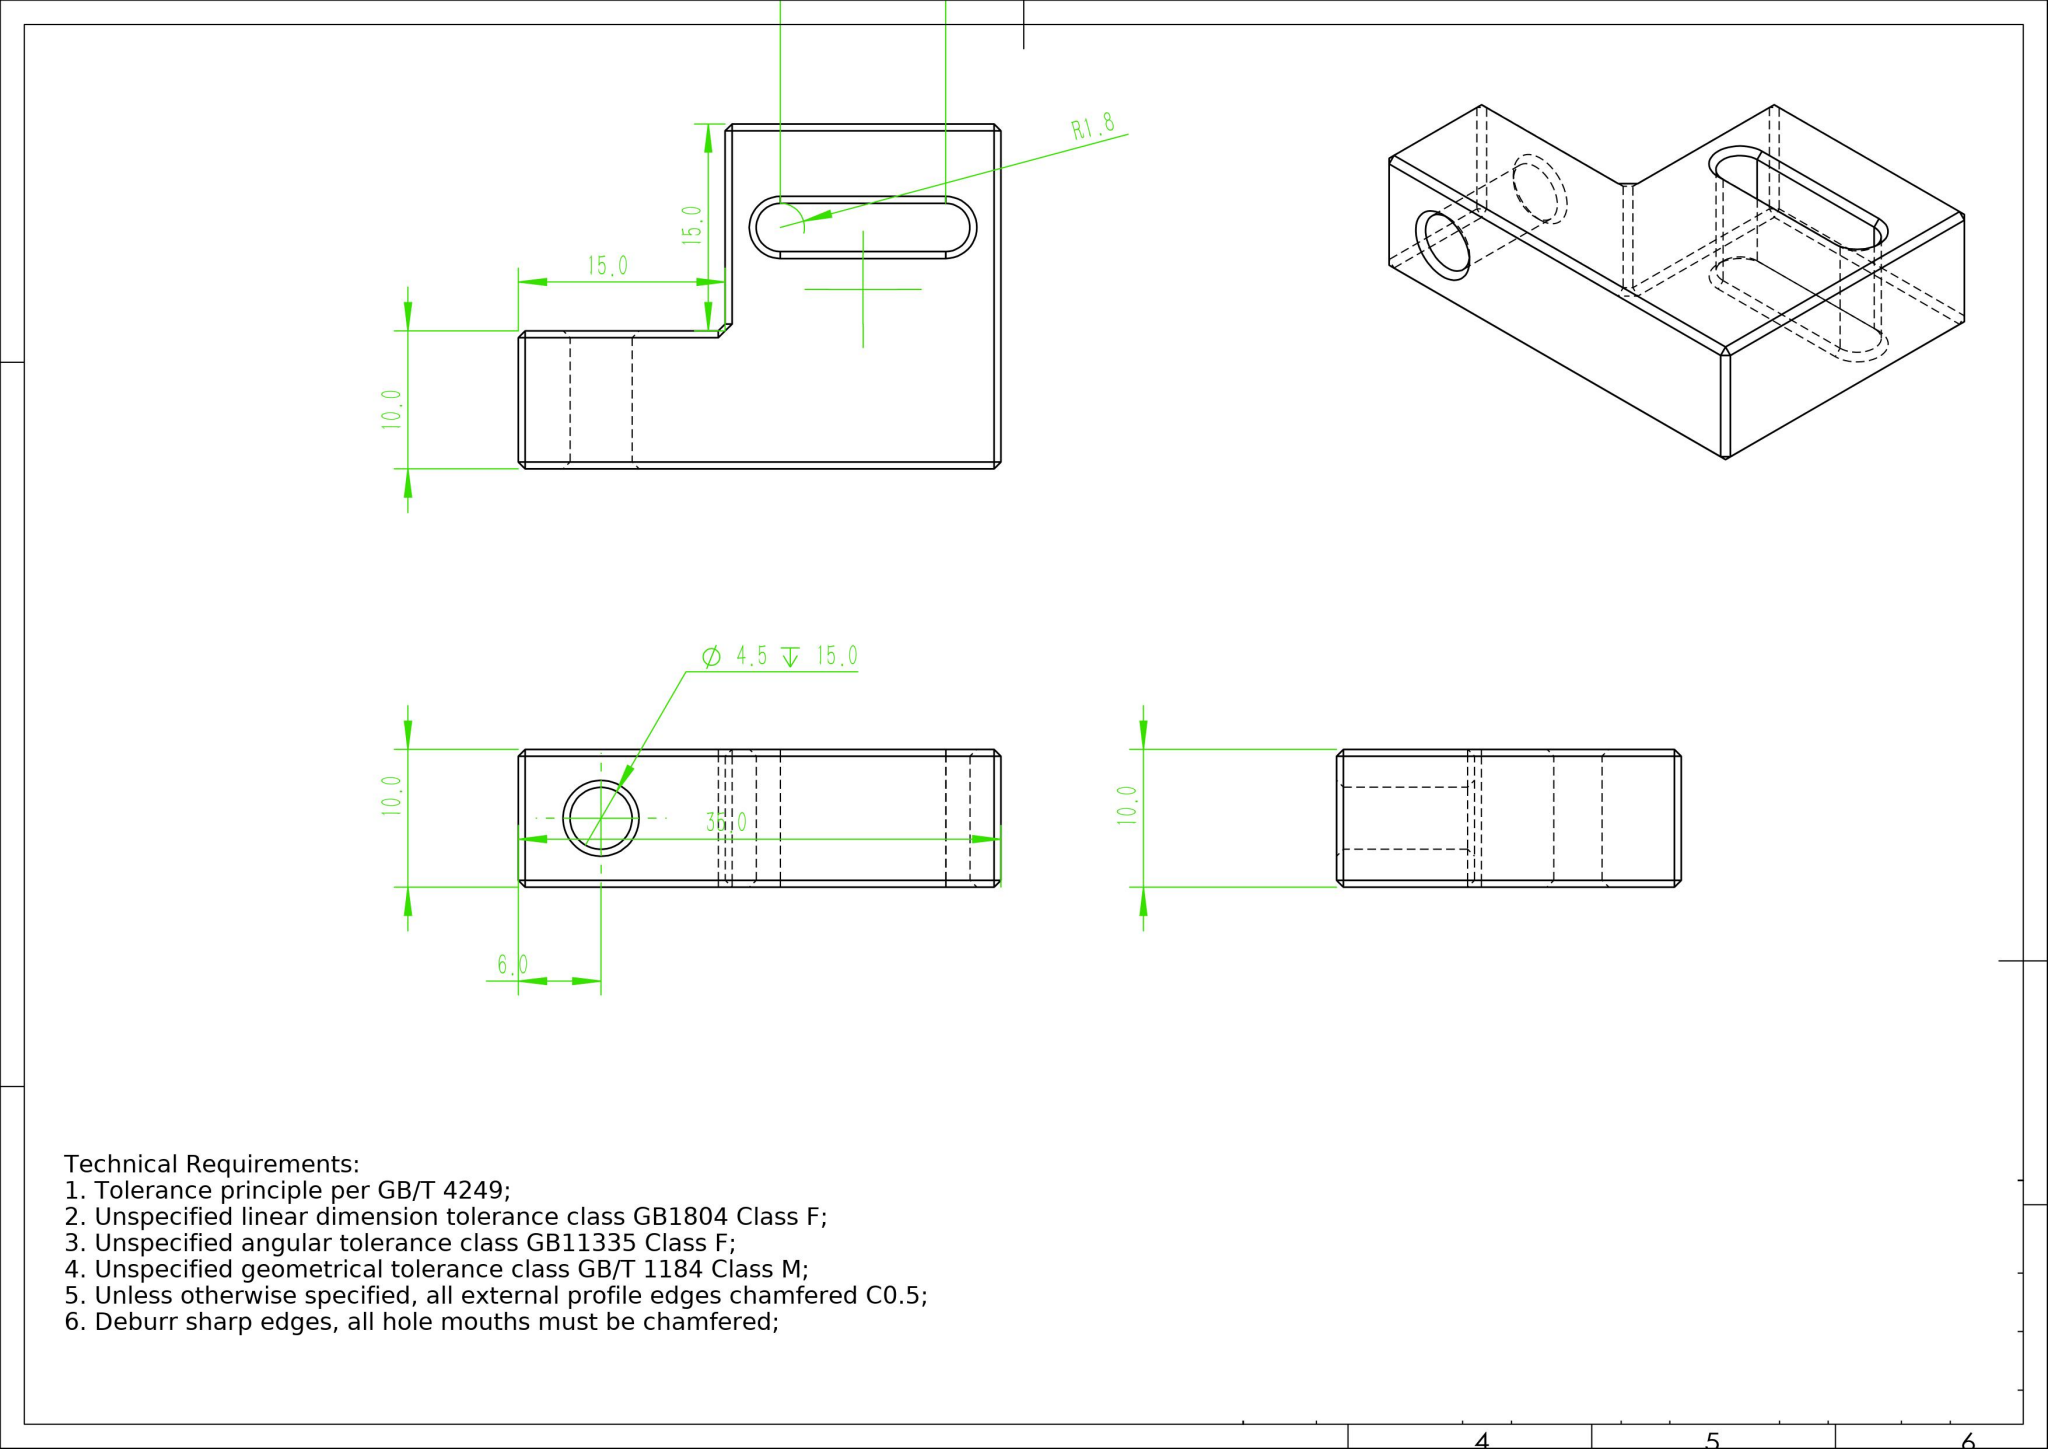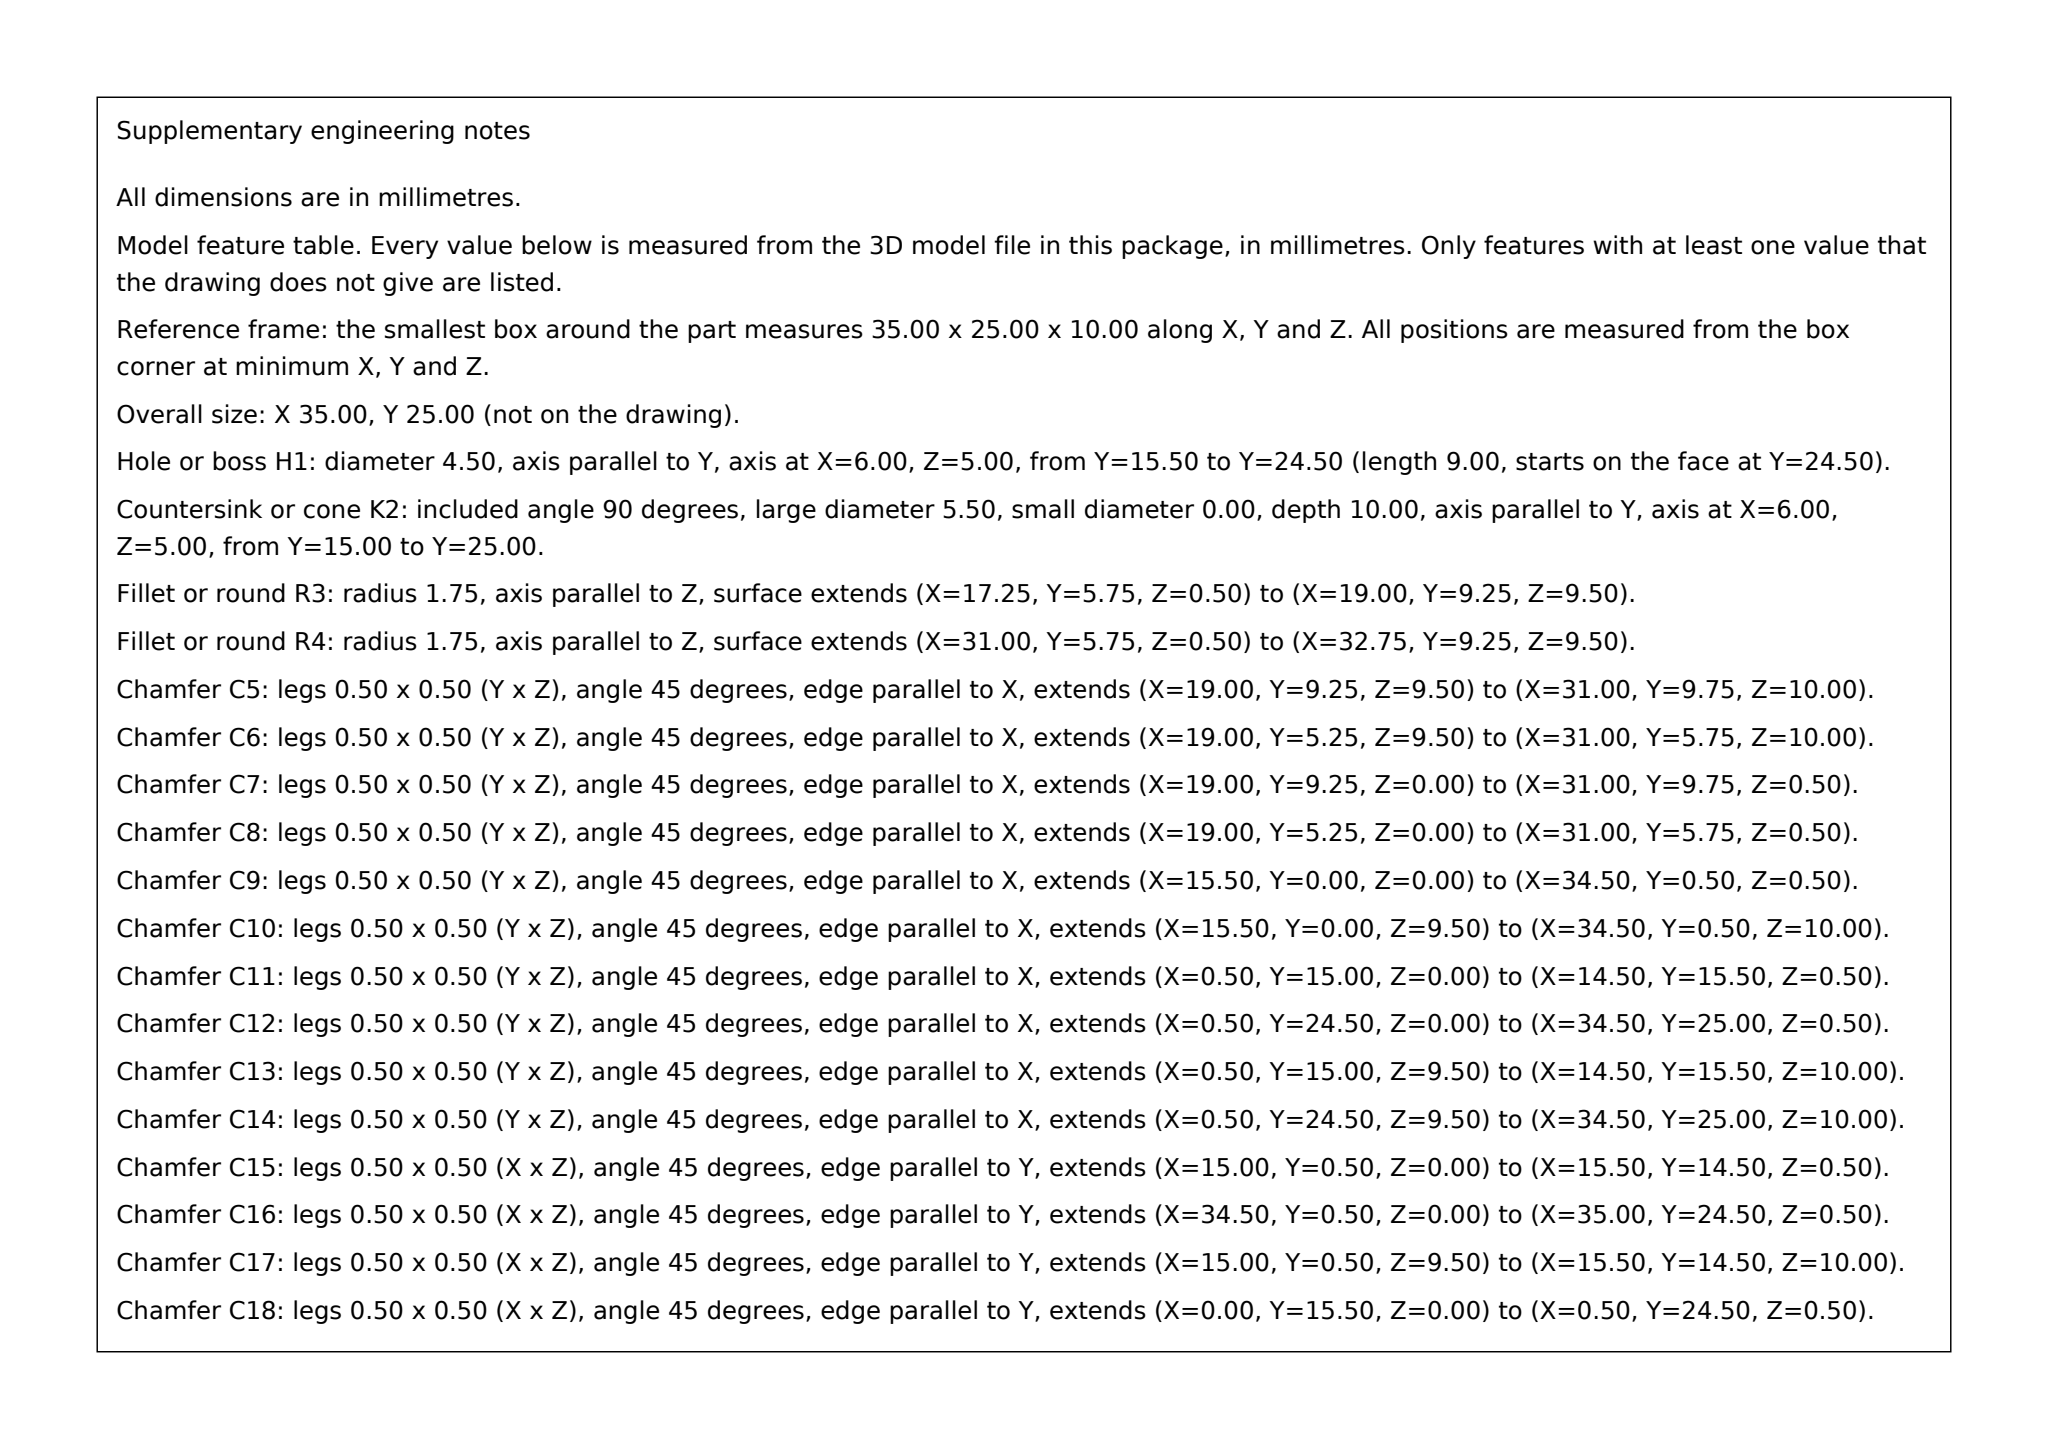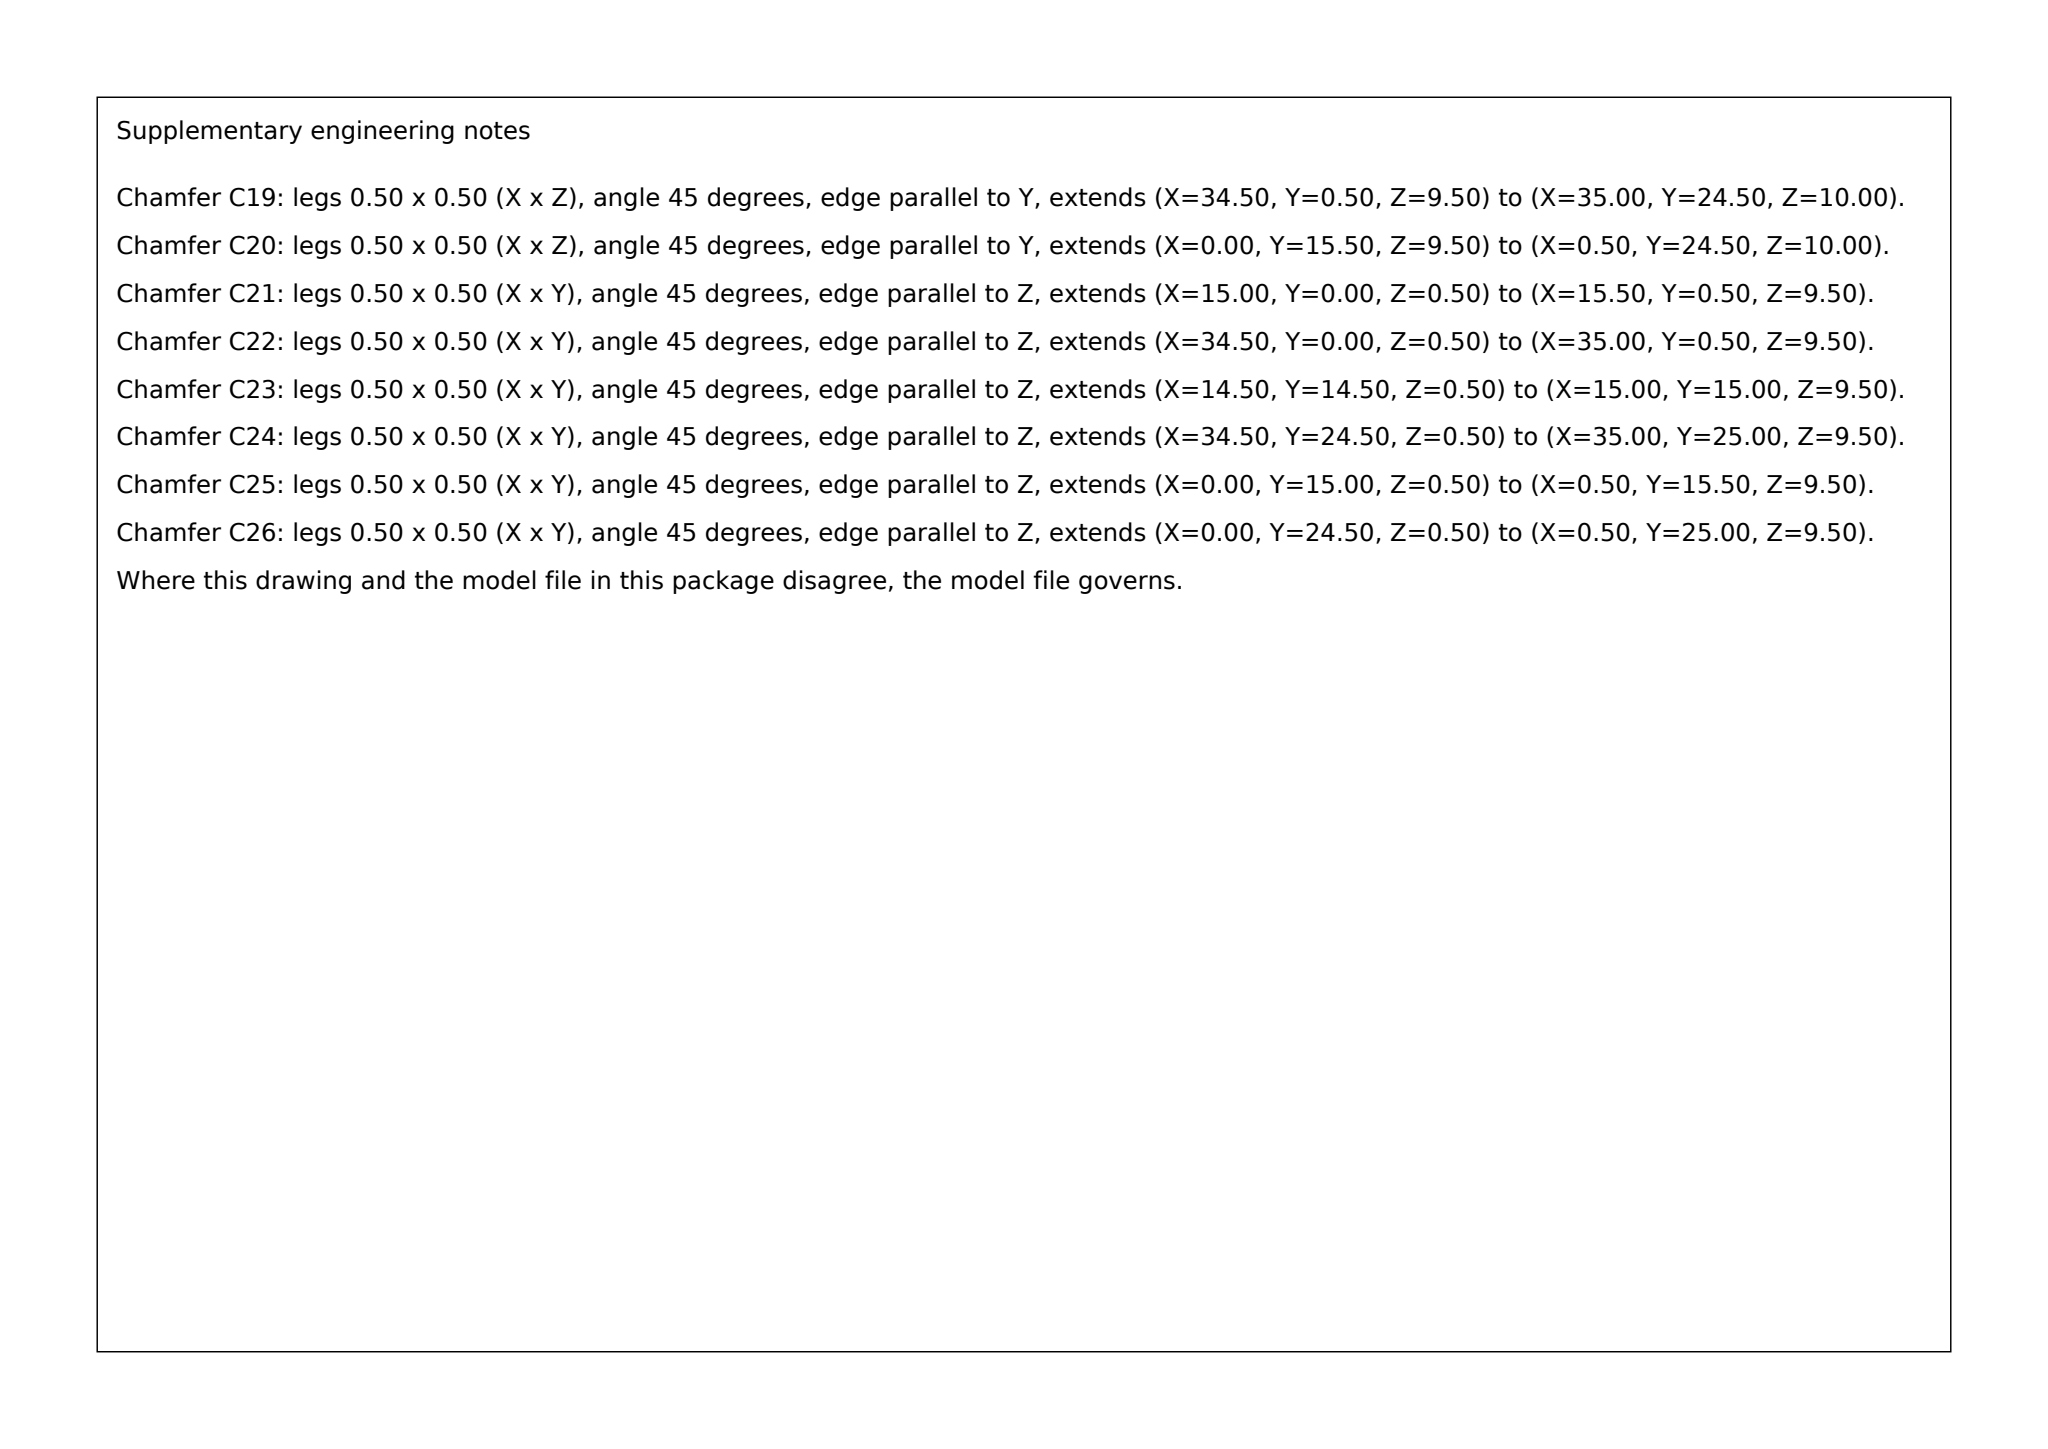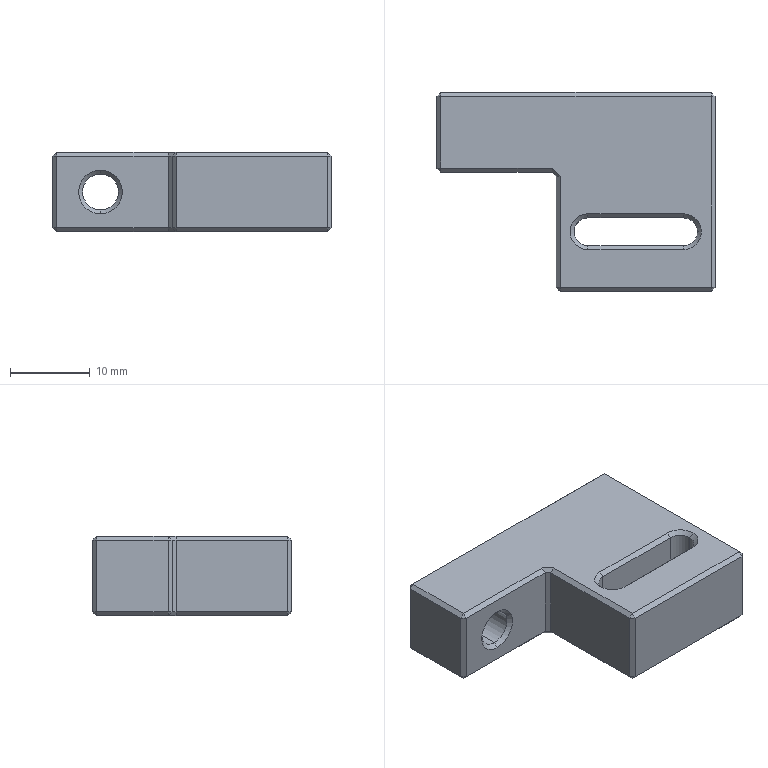Part | SolidWorks | mm | 1 solid | 59 faces | box 35 x 25 x 10 mm | volume 5778 mm3 | plane 44 | cone 10 | cylinder 5 | commonest cylinder face diameters 3.5 x3 4.5 x2
build123d program:
from build123d import *

# Parameters (mm, degrees)
SKETCH1_W                      = 50
SKETCH1_H                      = 25
BOSS_EXTRUDE1_DEPTH            = 10
SKETCH2_W                      = 30
SKETCH2_H                      = 15
CUT_EXTRUDE1_DEPTH             = 30.686
CUT_EXTRUDE2_DEPTH             = 30.686
SKETCH6_W                      = 15
SKETCH6_H                      = 10
CUT_EXTRUDE3_DEPTH             = 10
F_4_5_4_5_DIAMETER_HOLE2_D     = 4.5
F_4_5_4_5_DIAMETER_HOLE2_DEPTH = 15
F_4_5_4_5_DIAMETER_HOLE2_TIP   = 1.352
CHAMFER1_SIZE                  = 0.5


with BuildPart() as part:
    # Sketch1 → Boss-Extrude1 (new body)
    with BuildSketch(Plane.XY):
        Rectangle(SKETCH1_W, SKETCH1_H)
    extrude(amount=BOSS_EXTRUDE1_DEPTH)

    # Sketch2 → Cut-Extrude1 (cut, through all)
    with BuildSketch(Plane.XY.offset(10)):
        with Locations((-10, -5)):
            Rectangle(SKETCH2_W, SKETCH2_H)
    extrude(amount=-CUT_EXTRUDE1_DEPTH, mode=Mode.SUBTRACT)

    # Sketch3 → Cut-Extrude2 (cut, through all)
    with BuildSketch(Plane.XY.offset(10)):
        with BuildLine():
            Line((9, -3.25), (21, -3.25))
            ThreePointArc((21, -3.25), (22.75, -5), (21, -6.75))
            Line((21, -6.75), (9, -6.75))
            ThreePointArc((9, -6.75), (7.25, -5), (9, -3.25))
        make_face()
    extrude(amount=-CUT_EXTRUDE2_DEPTH, mode=Mode.SUBTRACT)

    # Sketch6 → Cut-Extrude3 (cut)
    with BuildSketch(Plane.XY.offset(10)):
        with Locations((-17.5, 7.5)):
            Rectangle(SKETCH6_W, SKETCH6_H)
    extrude(amount=-CUT_EXTRUDE3_DEPTH, mode=Mode.SUBTRACT)

    # 4.5 _4.5_ Diameter Hole2
    with Locations(Plane(origin=(0, 12.5, 0), x_dir=(1, 0, 0), z_dir=(0, 1, 0))):
        with Locations((-4, -5)):
            Hole(F_4_5_4_5_DIAMETER_HOLE2_D / 2, depth=F_4_5_4_5_DIAMETER_HOLE2_DEPTH)
            with Locations((0, 0, -(F_4_5_4_5_DIAMETER_HOLE2_DEPTH + F_4_5_4_5_DIAMETER_HOLE2_TIP / 2))):  # 118° drill point
                Cone(0, F_4_5_4_5_DIAMETER_HOLE2_D / 2, F_4_5_4_5_DIAMETER_HOLE2_TIP, mode=Mode.SUBTRACT)

    # Chamfer1
    chamfer1_edges = [part.edges().sort_by_distance(p)[0] for p in [
        (25, 0, 10),
        (15, -12.5, 0),
        (15, -12.5, 10),
        (7.5, 12.5, 10),
        (-2.5, 2.5, 0),
        (5, -5, 0),
        (5, 2.5, 5),
        (5, -12.5, 5),
        (5, -5, 10),
        (-2.5, 2.5, 10),
        (7.25, -5, 0),
        (15, -3.25, 0),
        (22.75, -5, 0),
        (15, -6.75, 0),
        (7.25, -5, 10),
        (15, -6.75, 10),
        (22.75, -5, 10),
        (15, -3.25, 10),
        (-10, 7.5, 0),
        (-10, 12.5, 5),
        (-10, 2.5, 5),
        (7.5, 12.5, 0),
        (-10, 7.5, 10),
        (25, 0, 0),
        (-1.75, 2.5, 5),
        (-1.75, 12.5, 5),
        (25, 12.5, 5),
        (25, -12.5, 5),
    ]]
    chamfer(chamfer1_edges, length=CHAMFER1_SIZE)


solid = part.part